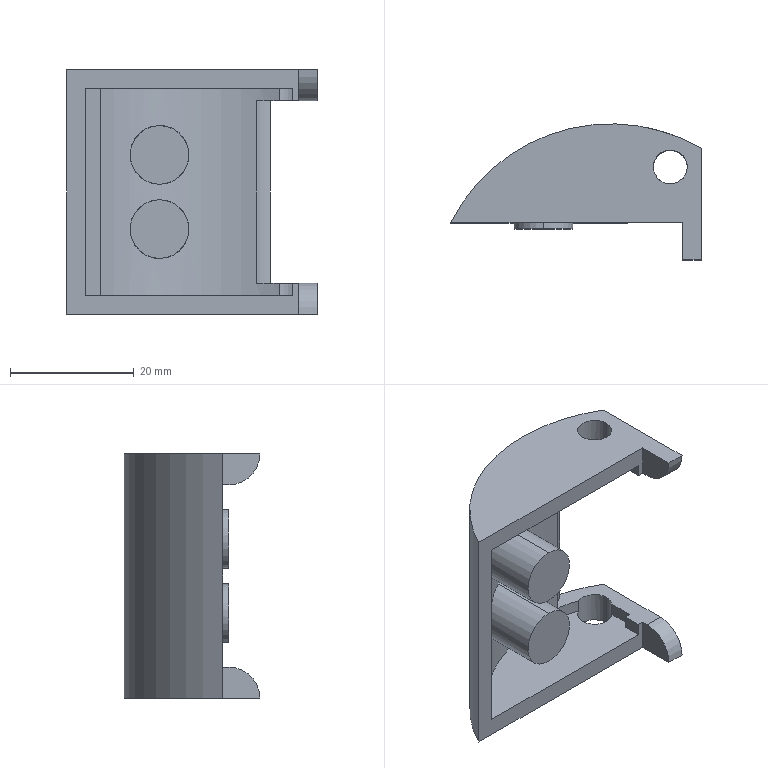Component | SolidWorks | Hinge2-2 | 1 solid | 35 faces | volume 8355 mm3 | plane 22 | cylinder 13 | commonest cylinder face diameters 9.5 x4 5.5 x4 10 x2 51.901 x1 57.901 x1 12 x1